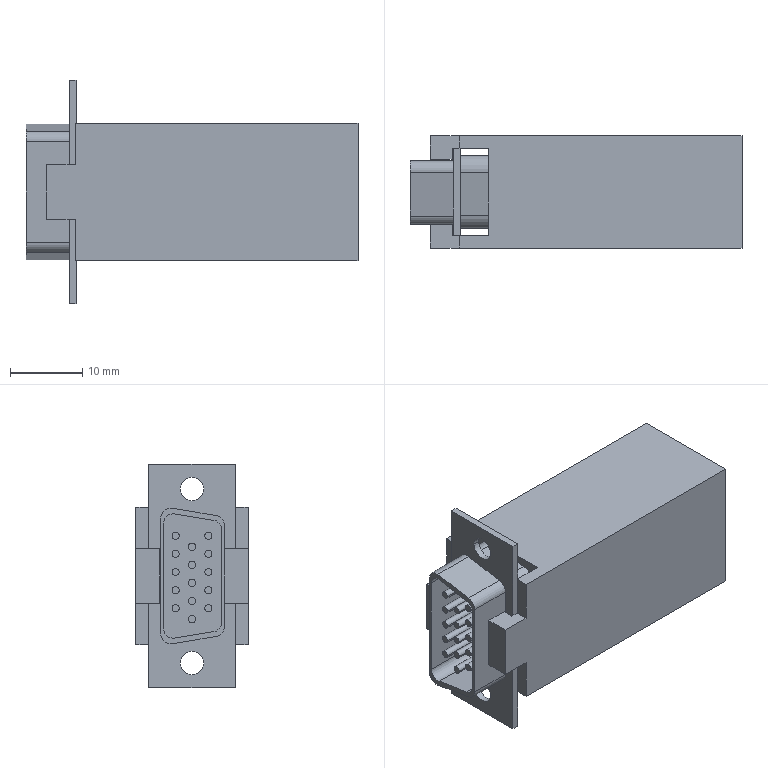Component | SolidWorks | F-SWS-005-000-000-1_F-SCHUNK-0301265 KAS-A15-A-1 | 1 solid | 106 faces | box 45.8 x 15.5 x 30.8 mm | volume 11655 mm3 | plane 60 | cylinder 46 | commonest cylinder face diameters 1 x30 3.2 x4 4 x4 2.794 x4 2.54 x4